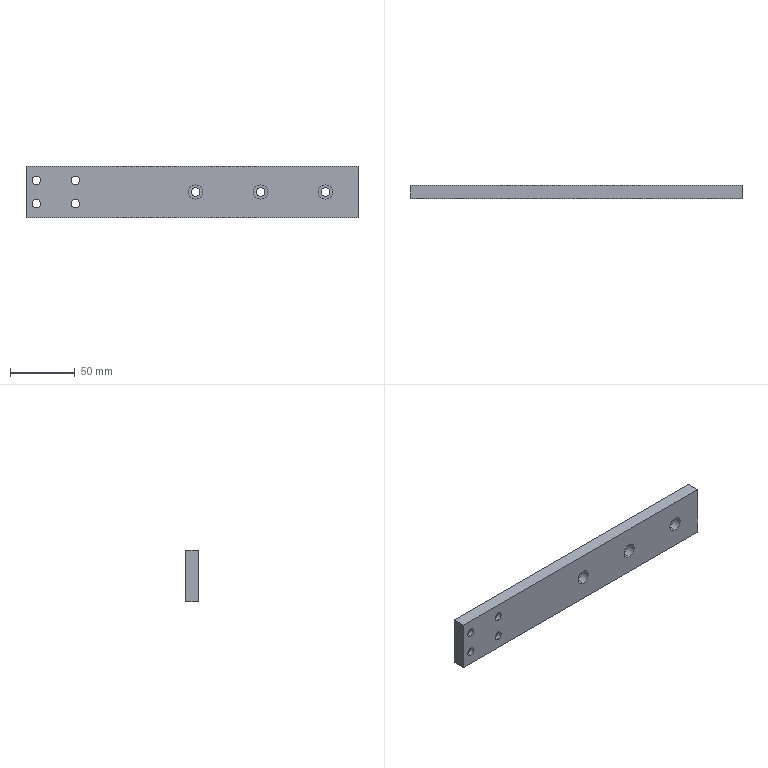Component | SolidWorks | 17081801-804-024A-1 | 1 solid | 53 faces | box 255.5 x 10 x 40 mm | volume 96167 mm3 | cylinder 34 | plane 13 | cone 6 | commonest cylinder face diameters 11 x14 6.6 x14 5 x6 | material AL6061
build123d program:
from build123d import *

# Parameters (mm, degrees)
SKETCH1_W                                       = 255.5
SKETCH1_H                                       = 40
BOSS_EXTRUDE1_DEPTH                             = 5
M6_HEX_SOCKET_HEAD_CAP_SCREW_CBORE1_D           = 6.6
M6_HEX_SOCKET_HEAD_CAP_SCREW_CBORE1_DEPTH       = 60
M6_HEX_SOCKET_HEAD_CAP_SCREW_CBORE1_CBORE_D     = 11
M6_HEX_SOCKET_HEAD_CAP_SCREW_CBORE1_CBORE_DEPTH = 6.4
M6_HEX_SOCKET_HEAD_CAP_SCREW_CBORE1_TIP         = 1.983
M6_TAPPED_HOLE1_D                               = 5
M6_TAPPED_HOLE1_DEPTH                           = 15
M6_TAPPED_HOLE1_TIP                             = 1.502
M6_HEX_SOCKET_HEAD_CAP_SCREW_CBORE2_D           = 6.6
M6_HEX_SOCKET_HEAD_CAP_SCREW_CBORE2_DEPTH       = 60
M6_HEX_SOCKET_HEAD_CAP_SCREW_CBORE2_CBORE_D     = 11
M6_HEX_SOCKET_HEAD_CAP_SCREW_CBORE2_CBORE_DEPTH = 6.4
M6_HEX_SOCKET_HEAD_CAP_SCREW_CBORE2_TIP         = 1.983


with BuildPart() as part:
    # Sketch1 → Boss-Extrude1 (new, symmetric)
    with BuildSketch(Plane(origin=(0, 0, 0), x_dir=(1, 0, 0), z_dir=(0, 1, 0))):
        Rectangle(SKETCH1_W, SKETCH1_H)
    extrude(amount=BOSS_EXTRUDE1_DEPTH, both=True)

    # M6 Hex Socket Head Cap Screw CBORE1
    with Locations(Plane(origin=(0, 5, 0), x_dir=(1, 0, 0), z_dir=(0, 1, 0))):
        with Locations((-89.75, 9), (-89.75, -9), (-119.75, 9), (-119.75, -9)):
            CounterBoreHole(M6_HEX_SOCKET_HEAD_CAP_SCREW_CBORE1_D / 2, M6_HEX_SOCKET_HEAD_CAP_SCREW_CBORE1_CBORE_D / 2, M6_HEX_SOCKET_HEAD_CAP_SCREW_CBORE1_CBORE_DEPTH, depth=M6_HEX_SOCKET_HEAD_CAP_SCREW_CBORE1_DEPTH)
            with Locations((0, 0, -(M6_HEX_SOCKET_HEAD_CAP_SCREW_CBORE1_DEPTH + M6_HEX_SOCKET_HEAD_CAP_SCREW_CBORE1_TIP / 2))):  # 118° drill point
                Cone(0, M6_HEX_SOCKET_HEAD_CAP_SCREW_CBORE1_D / 2, M6_HEX_SOCKET_HEAD_CAP_SCREW_CBORE1_TIP, mode=Mode.SUBTRACT)

    # M6 Tapped Hole1
    with Locations(Plane(origin=(127.75, 0, 0), x_dir=(0, 0, -1), z_dir=(1, 0, 0))):
        with Locations((15, 0), (0, 0), (-15, 0)):
            Hole(M6_TAPPED_HOLE1_D / 2, depth=M6_TAPPED_HOLE1_DEPTH)
            with Locations((0, 0, -(M6_TAPPED_HOLE1_DEPTH + M6_TAPPED_HOLE1_TIP / 2))):  # 118° drill point
                Cone(0, M6_TAPPED_HOLE1_D / 2, M6_TAPPED_HOLE1_TIP, mode=Mode.SUBTRACT)

    # M6 Hex Socket Head Cap Screw CBORE2
    with Locations(Plane(origin=(0, -5, 0), x_dir=(-1, 0, 0), z_dir=(0, -1, 0))):
        with Locations((-102.75, 0), (-52.75, 0), (-2.75, 0)):
            CounterBoreHole(M6_HEX_SOCKET_HEAD_CAP_SCREW_CBORE2_D / 2, M6_HEX_SOCKET_HEAD_CAP_SCREW_CBORE2_CBORE_D / 2, M6_HEX_SOCKET_HEAD_CAP_SCREW_CBORE2_CBORE_DEPTH, depth=M6_HEX_SOCKET_HEAD_CAP_SCREW_CBORE2_DEPTH)
            with Locations((0, 0, -(M6_HEX_SOCKET_HEAD_CAP_SCREW_CBORE2_DEPTH + M6_HEX_SOCKET_HEAD_CAP_SCREW_CBORE2_TIP / 2))):  # 118° drill point
                Cone(0, M6_HEX_SOCKET_HEAD_CAP_SCREW_CBORE2_D / 2, M6_HEX_SOCKET_HEAD_CAP_SCREW_CBORE2_TIP, mode=Mode.SUBTRACT)


solid = part.part

# Placed as in the assembly
solid = solid.moved(Location((109.25, 2105.4, 171), (0, 0, 0)))